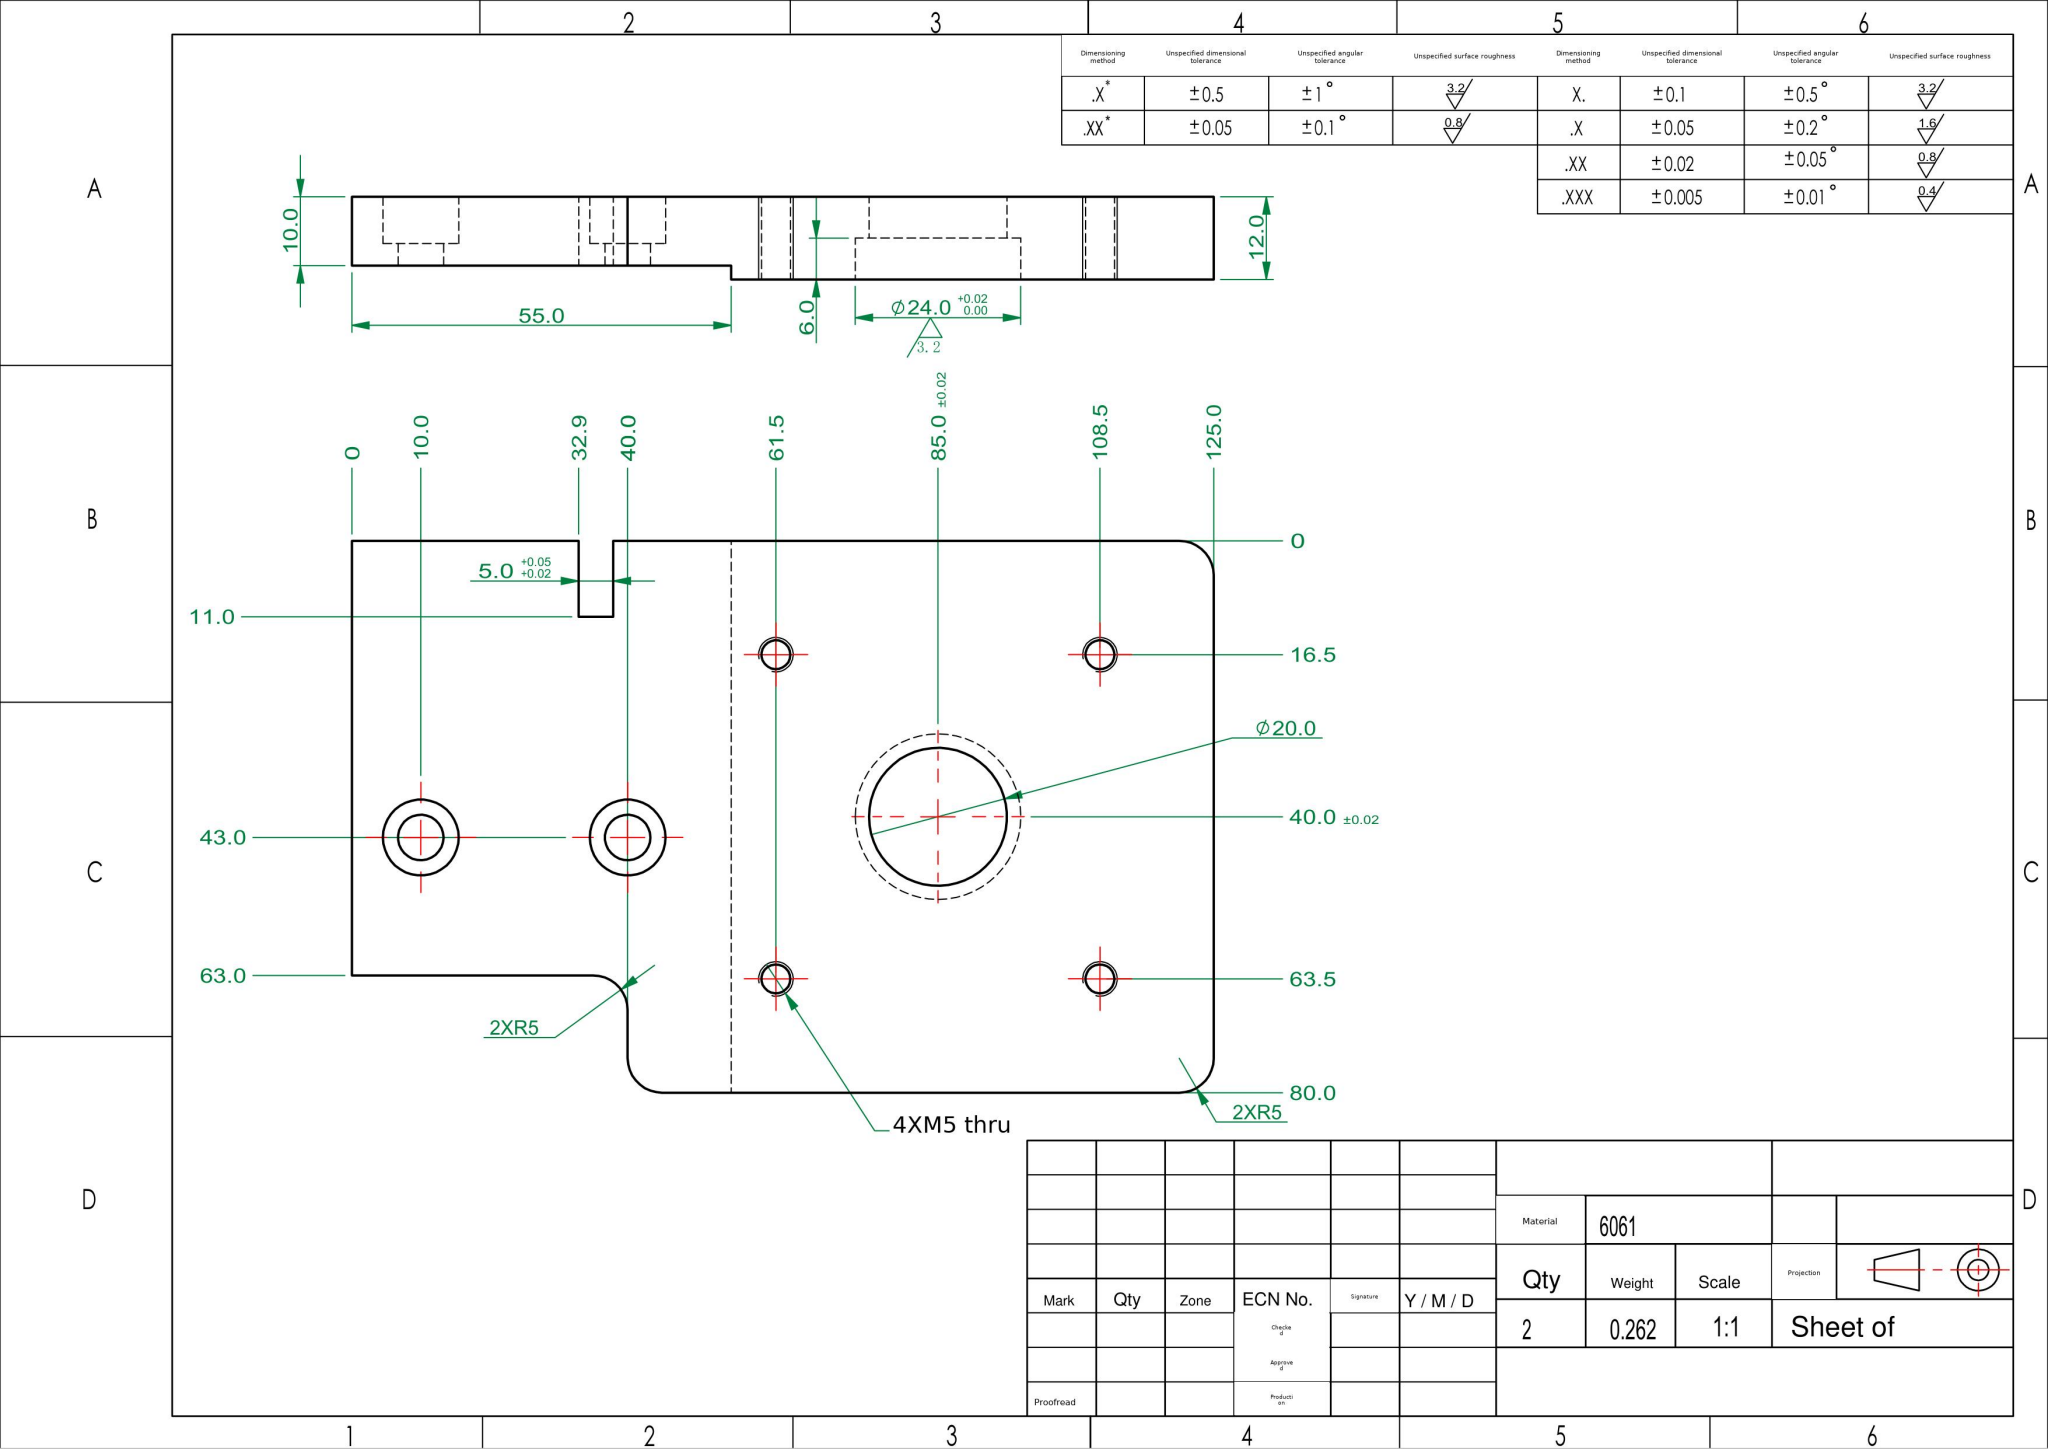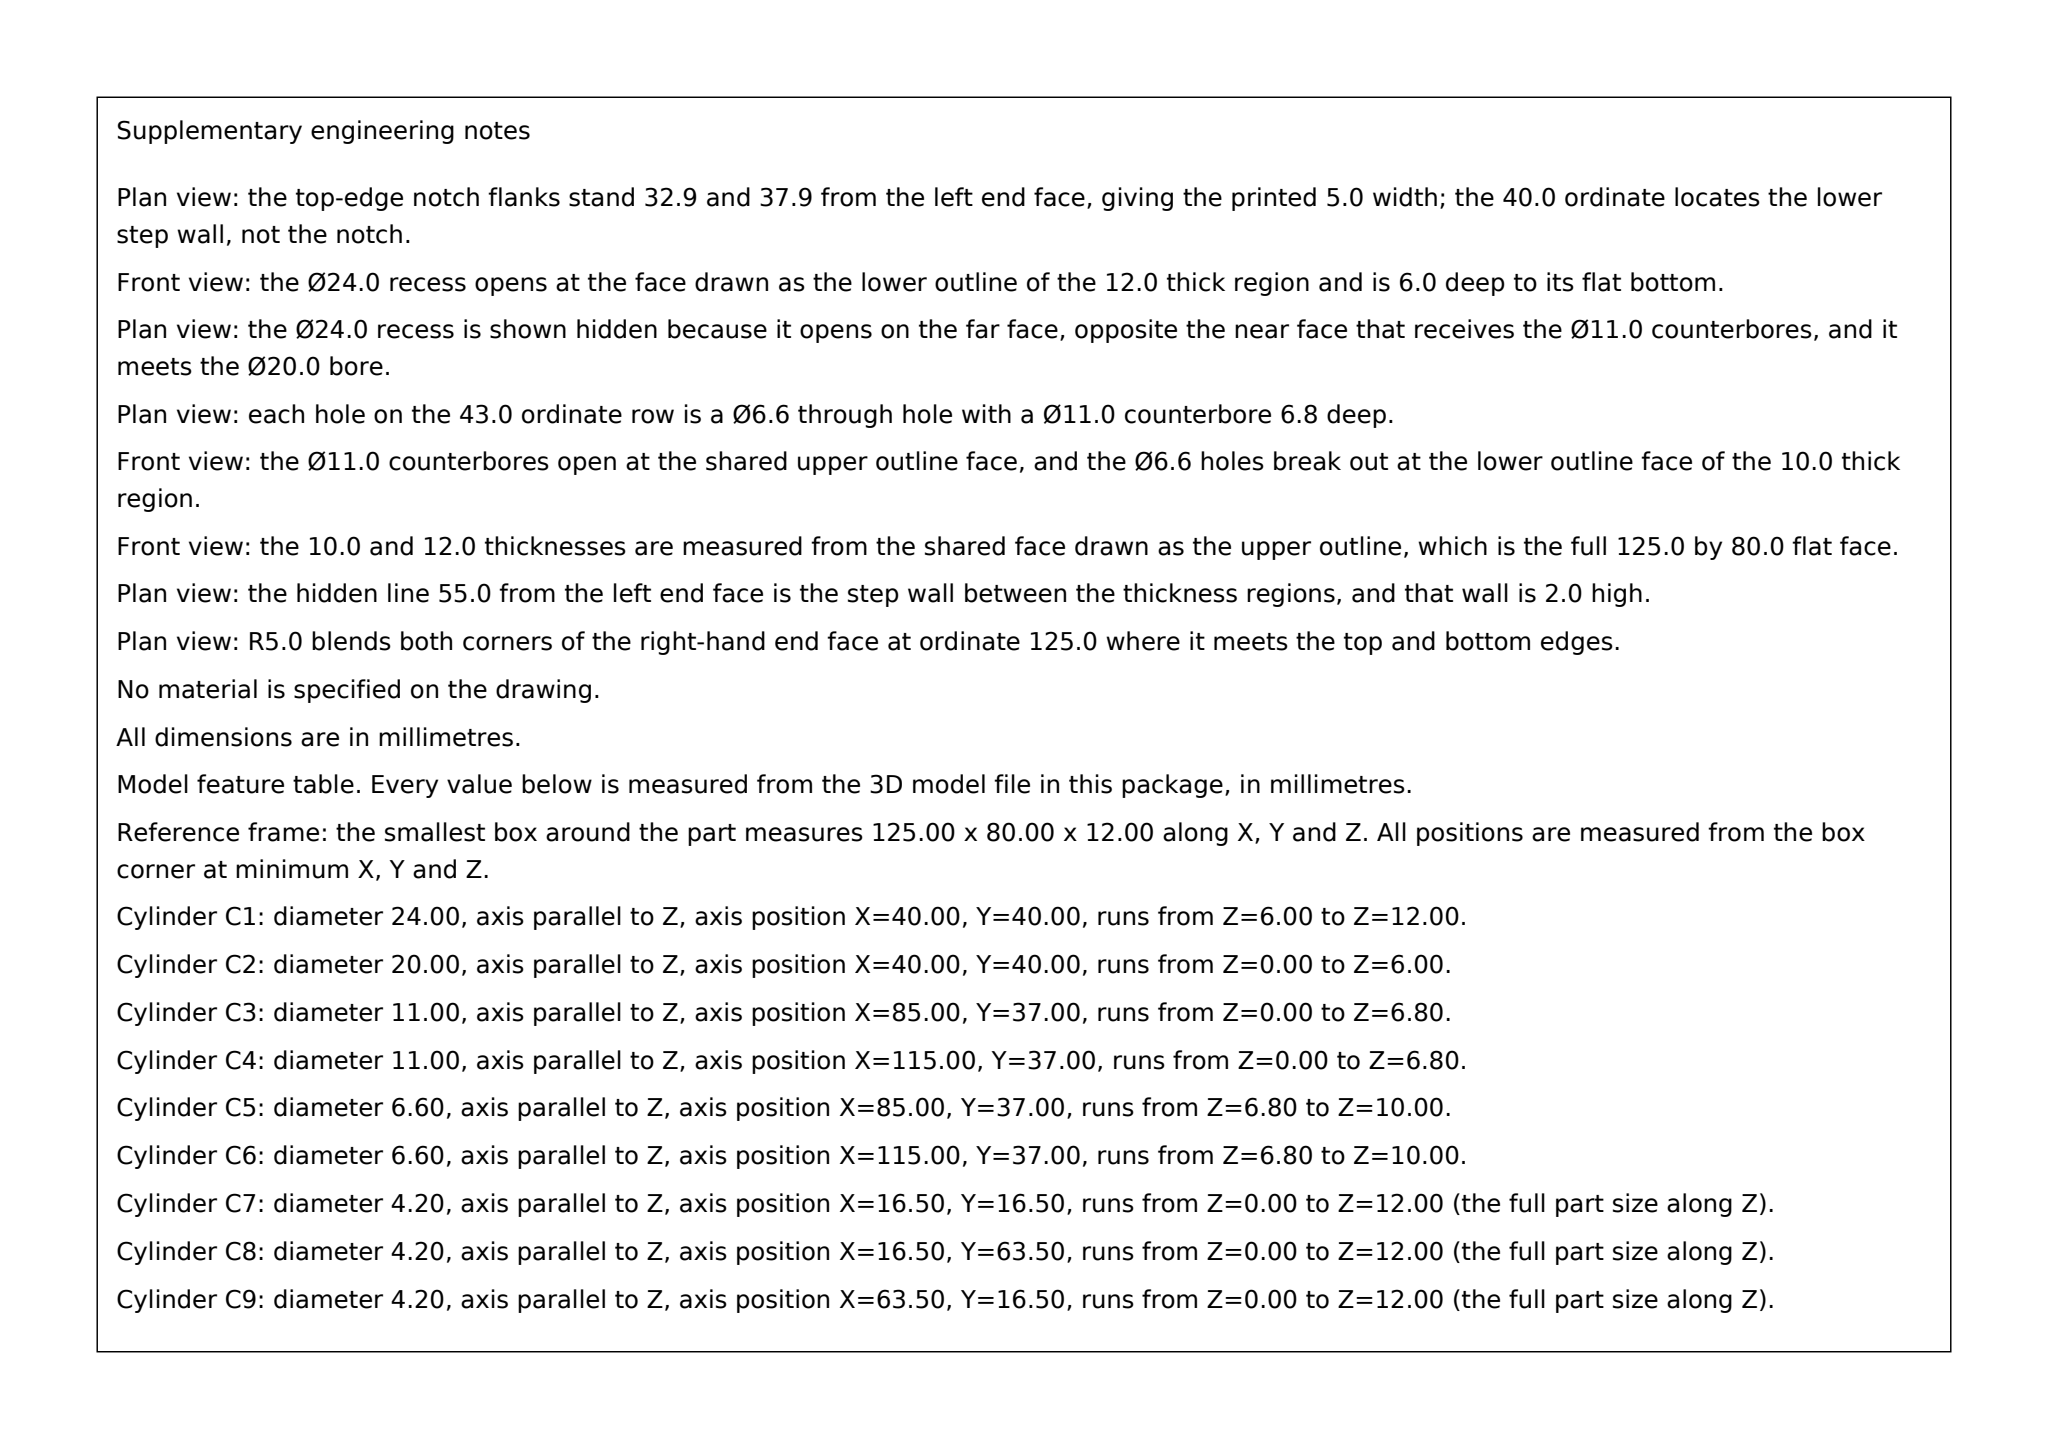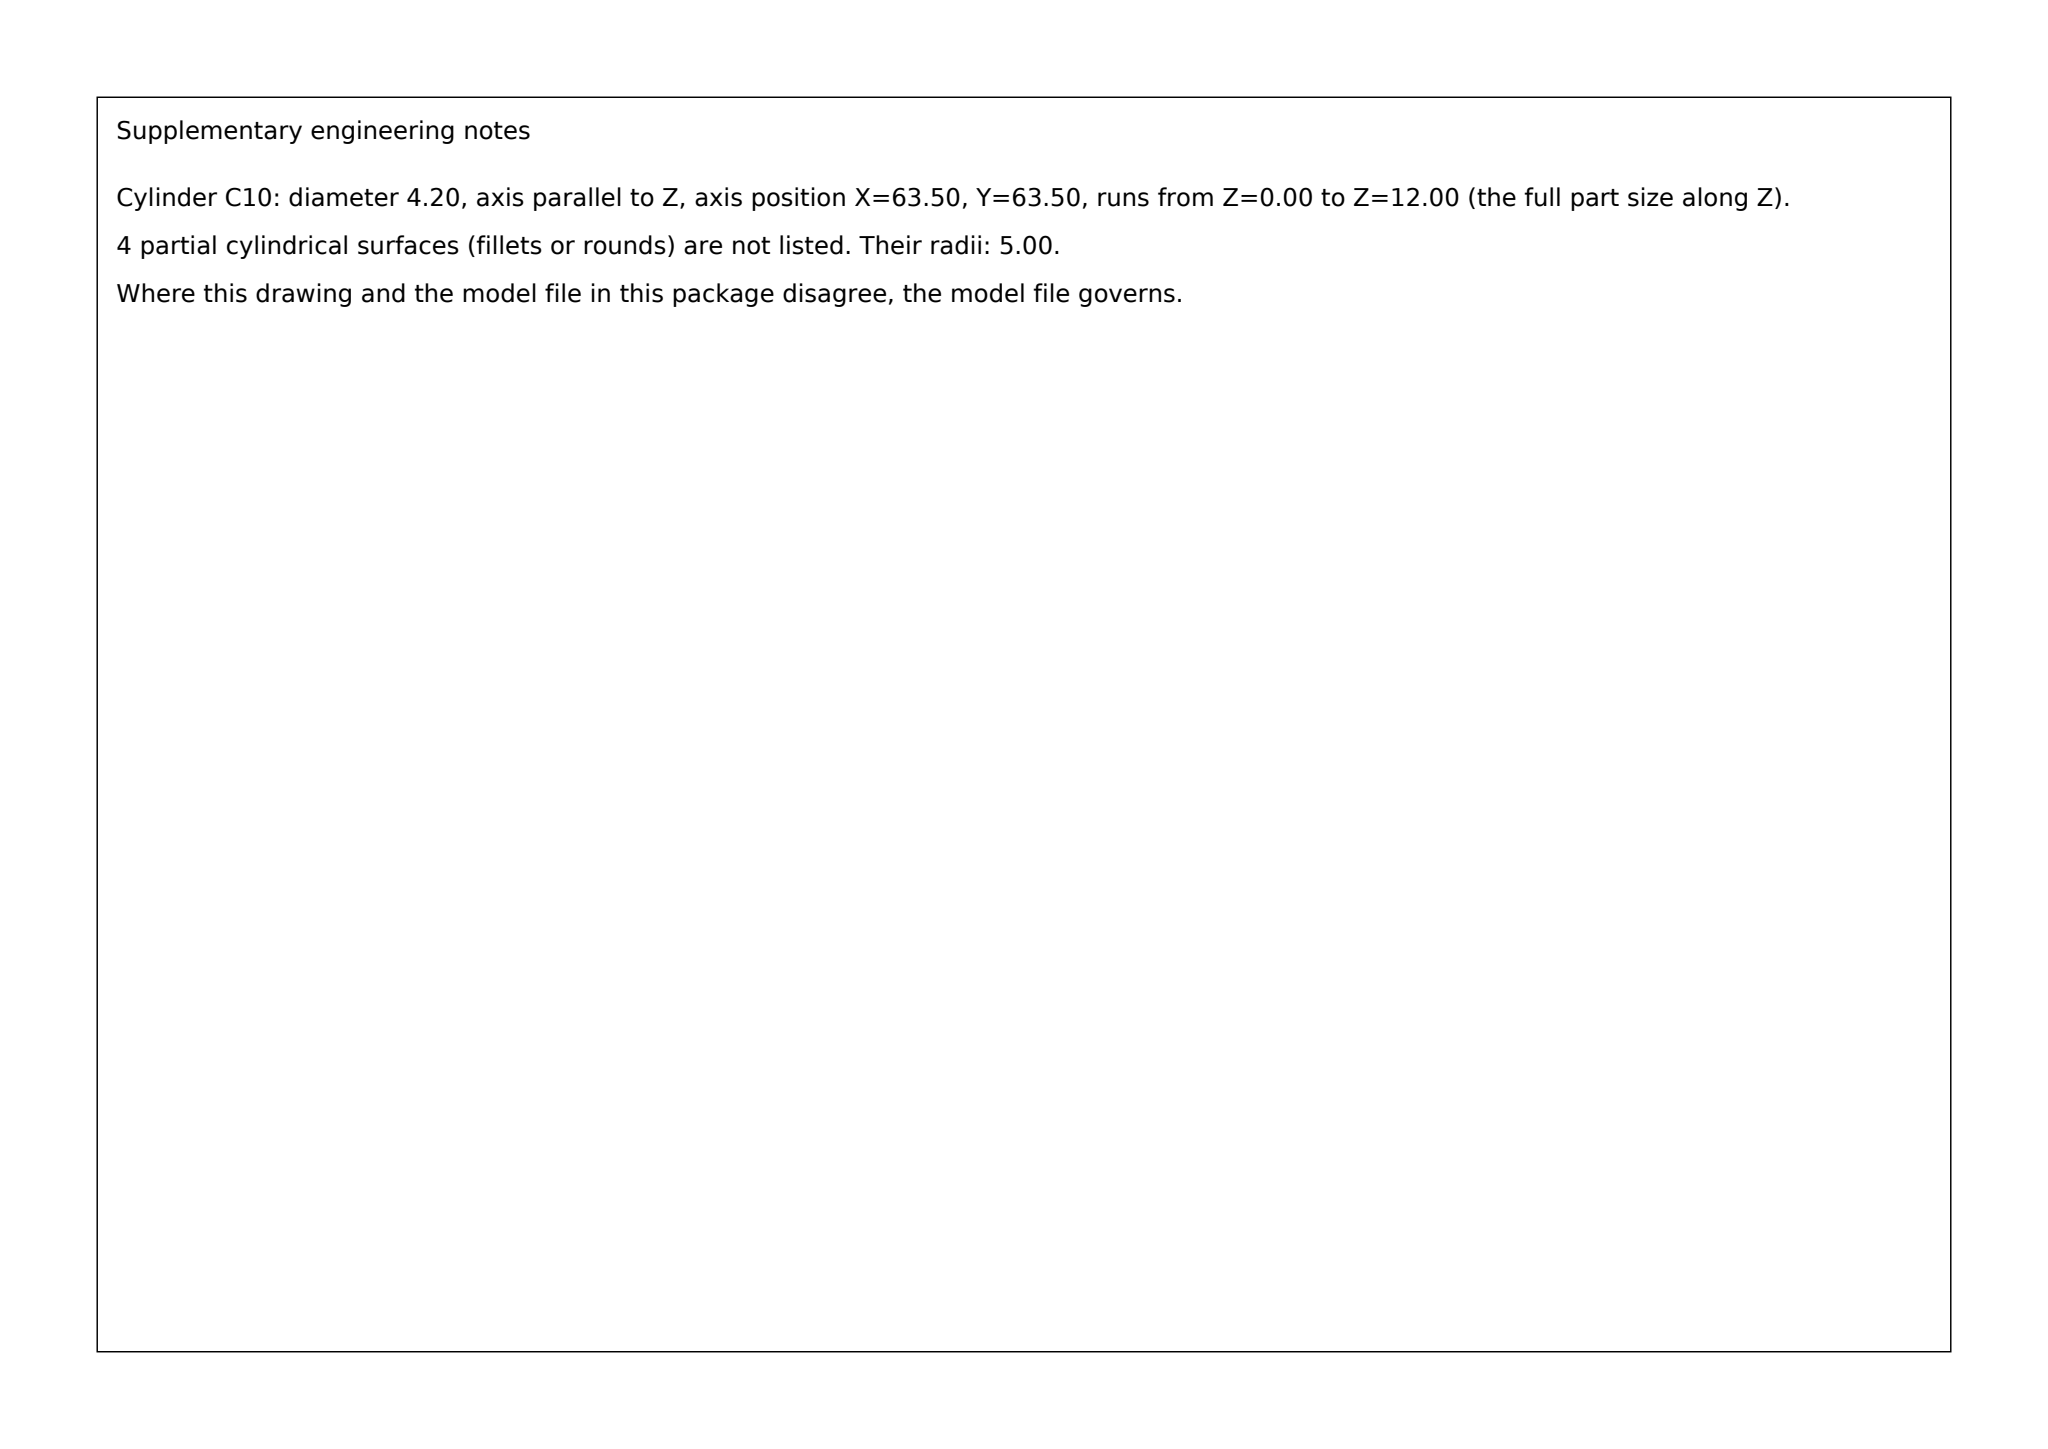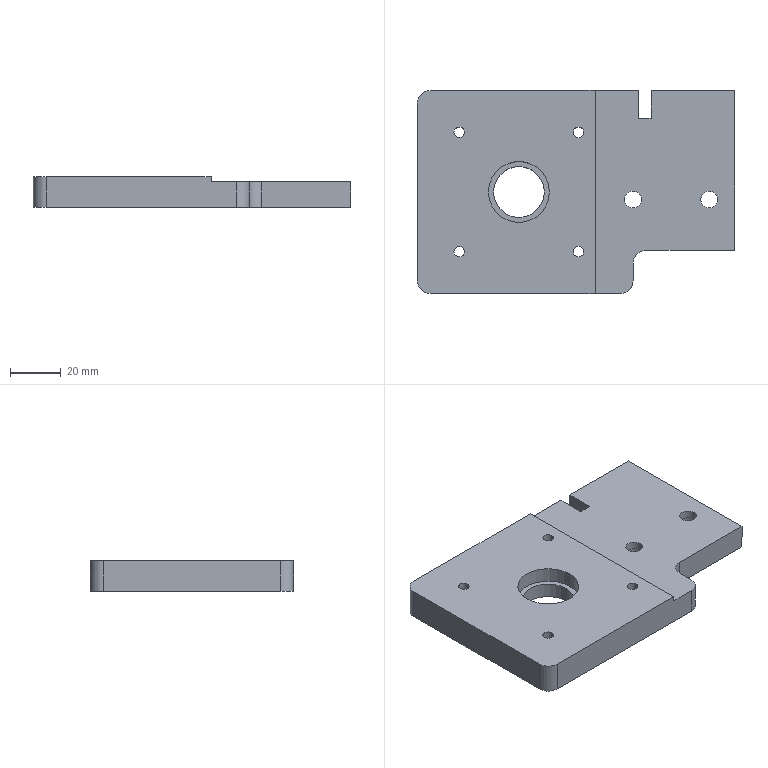Part | SolidWorks | mm | material 6061 | 1 solid | 41 faces | box 125 x 80 x 12 mm | volume 96946 mm3 | cylinder 24 | plane 17 | commonest cylinder face diameters 4.2 x8 11 x4 6.6 x4 10 x4 24 x2 20 x2
Drawing notes:
2X Ø6.6 THRU (holes on the 43.0 centerline, at X=10.0 and X=40.0 from the left edge datum) | from the solid: cylinders dia 6.6, axis z, at (85,37) and (115,37), length 3.2 (mirrored X: 125-115=10.0, 125-85=40.0; Y: 80-37=43.0)
2X CBORE Ø11.0 from top face, coaxial with the Ø6.6 holes at X=10.0 and X=40.0, Y=43.0 | from the solid: cylinders dia 11.0, axis z, at (85,37) and (115,37)
2X CBORE DEPTH 6.8 from top face (Ø11.0 counterbores at X=10.0 and X=40.0, Y=43.0) | from the solid: cylinders dia 11.0 length 6.8; axis plane z offset 6.8
ALL DIMENSIONS IN MILLIMETERS | from the solid: STEP model facts stated in mm
build123d program:
from build123d import *

# Parameters (mm, degrees)
SKETCH1_W                                         = 125
SKETCH1_H                                         = 80
BOSS_EXTRUDE1_DEPTH                               = 6
SKETCH2_R                                         = 10
CUT_EXTRUDE1_DEPTH                                = 46
SKETCH3_R                                         = 12
CUT_EXTRUDE2_DEPTH                                = 6
M5_TAPPED_HOLE1_D                                 = 4.2
SKETCH6_W                                         = 40
SKETCH6_H                                         = 17
CUT_EXTRUDE3_DEPTH                                = 23
SKETCH8_W                                         = 55
SKETCH8_H                                         = 80
CUT_EXTRUDE4_DEPTH                                = 2
HOLE_SIZE_ACCORDING_TO_HEXAGON_SOCKET_D           = 6.6
HOLE_SIZE_ACCORDING_TO_HEXAGON_SOCKET_CBORE_D     = 11
HOLE_SIZE_ACCORDING_TO_HEXAGON_SOCKET_CBORE_DEPTH = 6.8
FILLET1_R                                         = 5
SKETCH15_W                                        = 5
SKETCH15_H                                        = 22
CUT_EXTRUDE5_DEPTH                                = 28


with BuildPart() as part:
    # Sketch1 → Boss-Extrude1 (new, symmetric)
    with BuildSketch(Plane.XY):
        Rectangle(SKETCH1_W, SKETCH1_H)
    extrude(amount=BOSS_EXTRUDE1_DEPTH, both=True)

    # Sketch2 → Cut-Extrude1 (cut)
    with BuildSketch(Plane.XY.offset(6)):
        with Locations((-22.5, 0)):
            Circle(SKETCH2_R)
    extrude(amount=-CUT_EXTRUDE1_DEPTH, mode=Mode.SUBTRACT)

    # Sketch3 → Cut-Extrude2 (cut)
    with BuildSketch(Plane.XY.offset(6)):
        with Locations((-22.5, 0)):
            Circle(SKETCH3_R)
    extrude(amount=-CUT_EXTRUDE2_DEPTH, mode=Mode.SUBTRACT)

    # M5 Tapped Hole1 (through all)
    with Locations(Plane(origin=(1, 23.5, -6), x_dir=(-1, 0, 0), z_dir=(0, 0, -1))):
        with Locations((0, 0), (47, 0), (47, -47), (0, -47)):
            Hole(M5_TAPPED_HOLE1_D / 2)

    # Sketch6 → Cut-Extrude3 (cut)
    with BuildSketch(Plane(origin=(0, 0, -6), x_dir=(-1, 0, 0), z_dir=(0, 0, -1))):
        with Locations((-42.5, -31.5)):
            Rectangle(SKETCH6_W, SKETCH6_H)
    extrude(amount=-CUT_EXTRUDE3_DEPTH, mode=Mode.SUBTRACT)

    # Sketch8 → Cut-Extrude4 (cut)
    with BuildSketch(Plane.XY.offset(6)):
        with Locations((35, 0)):
            Rectangle(SKETCH8_W, SKETCH8_H)
    extrude(amount=-CUT_EXTRUDE4_DEPTH, mode=Mode.SUBTRACT)

    # Hole Size _ according to_ Hexagon Socket (through all)
    with Locations(Plane(origin=(52.5, -3, -6), x_dir=(-1, 0, 0), z_dir=(0, 0, -1))):
        with Locations((0, 0), (30, 0)):
            CounterBoreHole(HOLE_SIZE_ACCORDING_TO_HEXAGON_SOCKET_D / 2, HOLE_SIZE_ACCORDING_TO_HEXAGON_SOCKET_CBORE_D / 2, HOLE_SIZE_ACCORDING_TO_HEXAGON_SOCKET_CBORE_DEPTH)

    # Fillet1
    fillet1_edges = [part.edges().sort_by_distance(p)[0] for p in [
        (22.5, -40, -1),
        (22.5, -23, -1),
        (-62.5, -40, 0),
        (-62.5, 40, 0),
    ]]
    fillet(fillet1_edges, radius=FILLET1_R)

    # Sketch15 → Cut-Extrude5 (cut)
    with BuildSketch(Plane(origin=(0, 0, -6), x_dir=(-1, 0, 0), z_dir=(0, 0, -1))):
        with Locations((-27.1, 40)):
            Rectangle(SKETCH15_W, SKETCH15_H)
    extrude(amount=-CUT_EXTRUDE5_DEPTH, mode=Mode.SUBTRACT)


solid = part.part